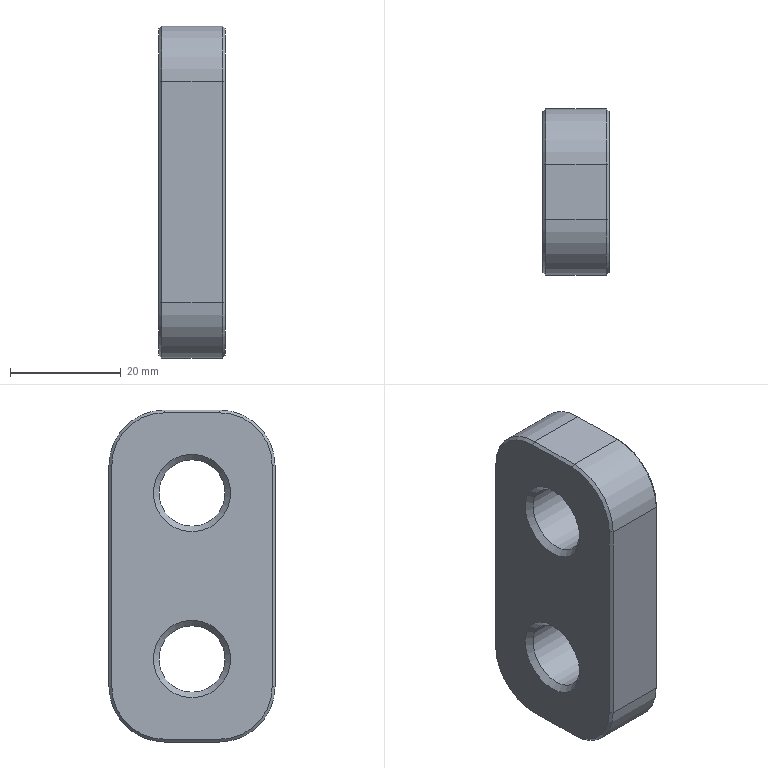Component | NX | SWIVEL_PLATE | 1 solid | 32 faces | volume 17736 mm3 | plane 14 | cone 12 | cylinder 6 | commonest cylinder face diameters 20 x4 12 x2